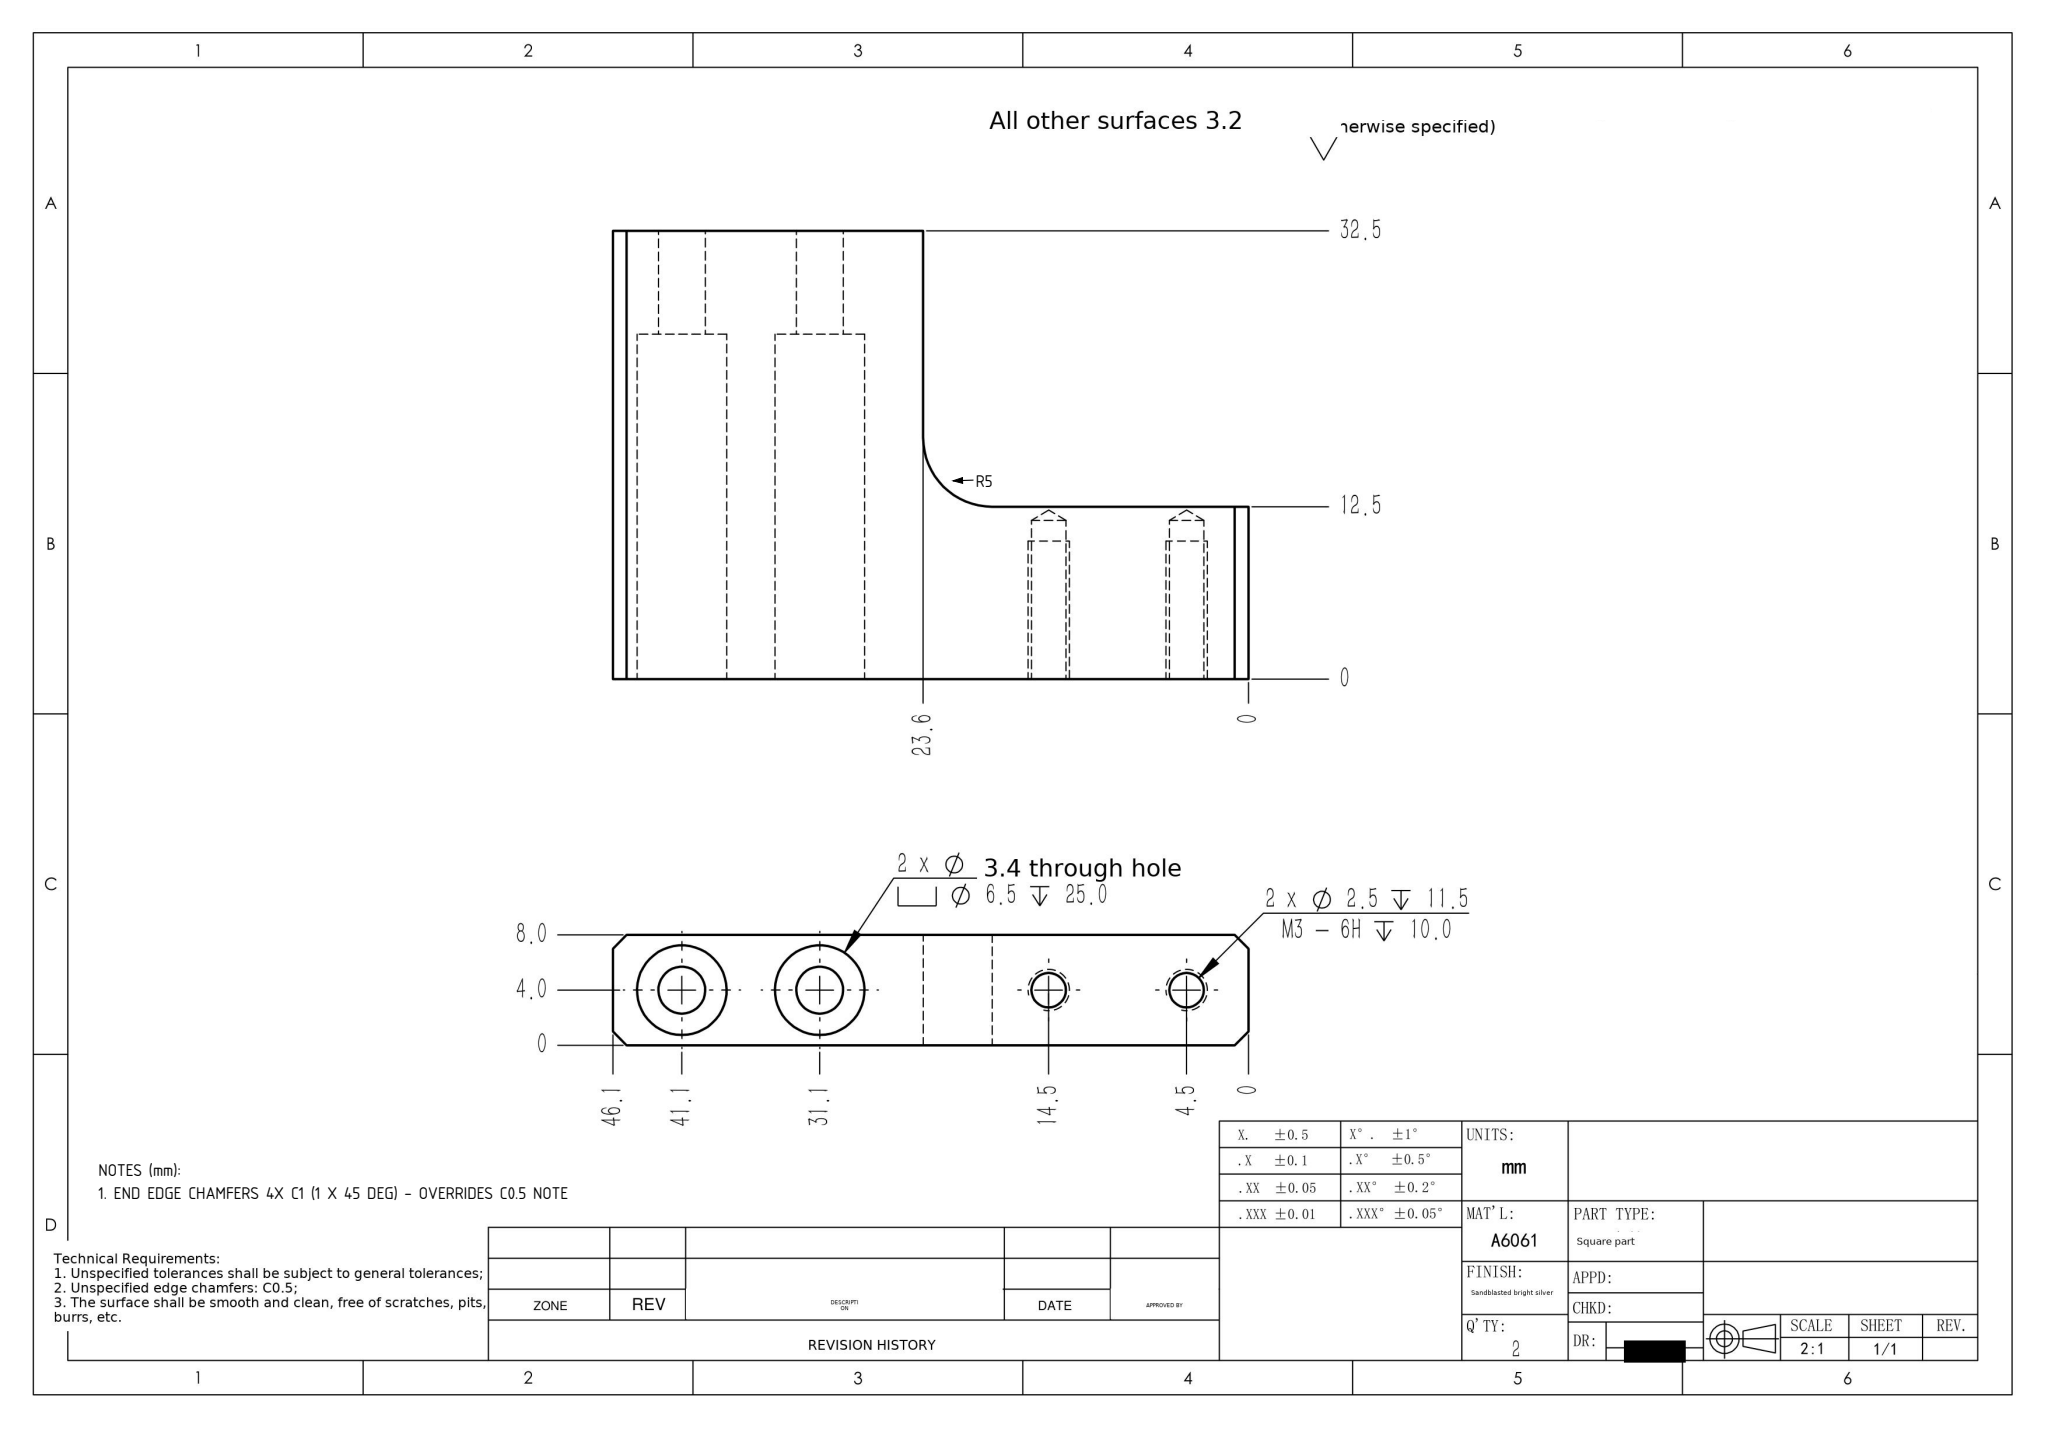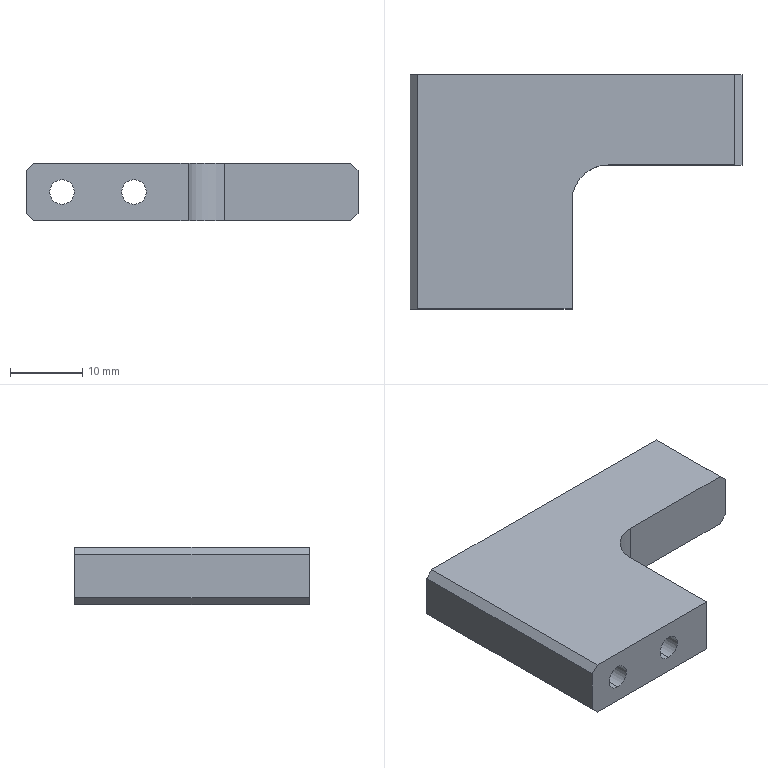Part | SolidWorks | mm | material A6061 | 1 solid | 31 faces | box 46.1 x 32.5 x 8 mm | volume 6297 mm3 | plane 14 | cylinder 13 | cone 4 | commonest cylinder face diameters 2.5 x4 6.5 x4 3.4 x4 10 x1
Drawing notes:
INNER CORNER FILLET R5 AT STEP TRANSITION, TANGENT TO VERTICAL FACE X=22.5 AND HORIZONTAL FACE Y=20.0 (ARC CENTER X27.5, Y15.0 FROM BBOX MIN CORNER), FULL 8.0 THICKNESS | from the solid: cylinders: [10.0, axis z, pos (27.5, 15.0), length 8.0] = R5 concave corner tangent to planes x=22.5 and y=20.0
END EDGE CHAMFERS 4X C1 (1 X 45 DEG) - OVERRIDES C0.5 NOTE | from the solid: inclined_planes: 4 faces at 45/90/45, size 1.0 x L x 1.0, at x=0 (z=0 & z=7, y 0-32.5) and x=45.1 (z=0 & z=7, y 20-32.5)
build123d program:
from build123d import *

# Parameters (mm, degrees)
SKETCH1_W                                       = 46.1
SKETCH1_H                                       = 32.5
BOSS_EXTRUDE1_DEPTH                             = 8
SKETCH2_W                                       = 23.6
SKETCH2_H                                       = 20
CUT_EXTRUDE1_DEPTH                              = 57.969
M3_HEX_SOCKET_HEAD_CAP_SCREW_CBORE1_D           = 3.4
M3_HEX_SOCKET_HEAD_CAP_SCREW_CBORE1_CBORE_D     = 6.5
M3_HEX_SOCKET_HEAD_CAP_SCREW_CBORE1_CBORE_DEPTH = 25
M3_TAPPED_HOLE1_D                               = 2.5
M3_TAPPED_HOLE1_DEPTH                           = 11.5
M3_TAPPED_HOLE1_TIP                             = 0.7511
FILLET1_R                                       = 5
CHAMFER1_SIZE                                   = 1


with BuildPart() as part:
    # Sketch1 → Boss-Extrude1 (new body)
    with BuildSketch(Plane.XY):
        with Locations((23.05, 16.25)):
            Rectangle(SKETCH1_W, SKETCH1_H)
    extrude(amount=BOSS_EXTRUDE1_DEPTH)

    # Sketch2 → Cut-Extrude1 (cut, through all)
    with BuildSketch(Plane.XY.offset(8)):
        with Locations((34.3, 10)):
            Rectangle(SKETCH2_W, SKETCH2_H)
    extrude(amount=-CUT_EXTRUDE1_DEPTH, mode=Mode.SUBTRACT)

    # M3 Hex Socket Head Cap Screw CBORE1 (through all)
    with Locations(Plane(origin=(0, 32.5, 0), x_dir=(1, 0, 0), z_dir=(0, 1, 0))):
        with Locations((5, -4), (15, -4)):
            CounterBoreHole(M3_HEX_SOCKET_HEAD_CAP_SCREW_CBORE1_D / 2, M3_HEX_SOCKET_HEAD_CAP_SCREW_CBORE1_CBORE_D / 2, M3_HEX_SOCKET_HEAD_CAP_SCREW_CBORE1_CBORE_DEPTH)

    # M3 Tapped Hole1
    with Locations(Plane(origin=(0, 32.5, 0), x_dir=(1, 0, 0), z_dir=(0, 1, 0))):
        with Locations((41.6, -4), (31.6, -4)):
            Hole(M3_TAPPED_HOLE1_D / 2, depth=M3_TAPPED_HOLE1_DEPTH)
            with Locations((0, 0, -(M3_TAPPED_HOLE1_DEPTH + M3_TAPPED_HOLE1_TIP / 2))):  # 118° drill point
                Cone(0, M3_TAPPED_HOLE1_D / 2, M3_TAPPED_HOLE1_TIP, mode=Mode.SUBTRACT)

    # Fillet1
    fillet1_edges = [part.edges().sort_by_distance(p)[0] for p in [
        (22.5, 20, 4),
    ]]
    fillet(fillet1_edges, radius=FILLET1_R)

    # Chamfer1
    chamfer1_edges = [part.edges().sort_by_distance(p)[0] for p in [
        (46.1, 26.25, 0),
        (46.1, 26.25, 8),
        (0, 16.25, 8),
        (0, 16.25, 0),
    ]]
    chamfer(chamfer1_edges, length=CHAMFER1_SIZE)


solid = part.part
STEP:
#1=CARTESIAN_POINT('',(41.6,21.,2.75));
#2=VERTEX_POINT('',#1);
#3=CARTESIAN_POINT('',(41.6,21.,5.25));
#4=VERTEX_POINT('',#3);
#5=CARTESIAN_POINT('',(41.6,21.,4.));
#6=DIRECTION('',(0.,1.,0.));
#7=DIRECTION('',(0.,0.,1.));
#8=AXIS2_PLACEMENT_3D('',#5,#6,#7);
#9=CIRCLE('',#8,1.25);
#10=EDGE_CURVE('',#2,#4,#9,.T.);
#11=ORIENTED_EDGE('',*,*,#10,.F.);
#12=CARTESIAN_POINT('',(41.6,32.5,2.75));
#13=VERTEX_POINT('',#12);
#14=CARTESIAN_POINT('',(41.6,32.5,2.75));
#15=DIRECTION('',(0.,1.,0.));
#16=VECTOR('',#15,1000.);
#17=LINE('',#14,#16);
#18=EDGE_CURVE('',#2,#13,#17,.T.);
#19=ORIENTED_EDGE('',*,*,#18,.T.);
#20=CARTESIAN_POINT('',(41.6,32.5,5.25));
#21=VERTEX_POINT('',#20);
#22=CARTESIAN_POINT('',(41.6,32.5,4.));
#23=DIRECTION('',(0.,1.,0.));
#24=DIRECTION('',(0.,0.,1.));
#25=AXIS2_PLACEMENT_3D('',#22,#23,#24);
#26=CIRCLE('',#25,1.25);
#27=EDGE_CURVE('',#13,#21,#26,.T.);
#28=ORIENTED_EDGE('',*,*,#27,.T.);
#29=CARTESIAN_POINT('',(41.6,32.5,5.25));
#30=DIRECTION('',(0.,1.,0.));
#31=VECTOR('',#30,1000.);
#32=LINE('',#29,#31);
#33=EDGE_CURVE('',#4,#21,#32,.T.);
#34=ORIENTED_EDGE('',*,*,#33,.F.);
#35=EDGE_LOOP('',(#11,#19,#28,#34));
#36=FACE_OUTER_BOUND('',#35,.T.);
#37=CARTESIAN_POINT('',(41.6,32.5,4.));
#38=DIRECTION('',(0.,1.,0.));
#39=DIRECTION('',(0.,0.,1.));
#40=AXIS2_PLACEMENT_3D('',#37,#38,#39);
#41=CYLINDRICAL_SURFACE('',#40,1.25);
#42=ADVANCED_FACE('',(#36),#41,.F.);
#43=CARTESIAN_POINT('',(41.6,20.249,4.));
#44=VERTEX_POINT('',#43);
#45=CARTESIAN_POINT('',(41.6,21.,5.25));
#46=DIRECTION('',(0.,0.515,0.8572));
#47=VECTOR('',#46,1000.);
#48=LINE('',#45,#47);
#49=EDGE_CURVE('',#44,#4,#48,.T.);
#50=ORIENTED_EDGE('',*,*,#49,.F.);
#51=CARTESIAN_POINT('',(41.6,21.,2.75));
#52=DIRECTION('',(0.,0.515,-0.8572));
#53=VECTOR('',#52,1000.);
#54=LINE('',#51,#53);
#55=EDGE_CURVE('',#44,#2,#54,.T.);
#56=ORIENTED_EDGE('',*,*,#55,.T.);
#57=ORIENTED_EDGE('',*,*,#10,.T.);
#58=EDGE_LOOP('',(#50,#56,#57));
#59=FACE_OUTER_BOUND('',#58,.T.);
#60=CARTESIAN_POINT('',(41.6,21.,4.));
#61=DIRECTION('',(0.,1.,0.));
#62=DIRECTION('',(0.,0.,1.));
#63=AXIS2_PLACEMENT_3D('',#60,#61,#62);
#64=CONICAL_SURFACE('',#63,1.25,1.03);
#65=ADVANCED_FACE('',(#59),#64,.F.);
#66=CARTESIAN_POINT('',(31.6,21.,2.75));
#67=VERTEX_POINT('',#66);
#68=CARTESIAN_POINT('',(31.6,21.,5.25));
#69=VERTEX_POINT('',#68);
#70=CARTESIAN_POINT('',(31.6,21.,4.));
#71=DIRECTION('',(0.,1.,0.));
#72=DIRECTION('',(0.,0.,1.));
#73=AXIS2_PLACEMENT_3D('',#70,#71,#72);
#74=CIRCLE('',#73,1.25);
#75=EDGE_CURVE('',#67,#69,#74,.T.);
#76=ORIENTED_EDGE('',*,*,#75,.F.);
#77=CARTESIAN_POINT('',(31.6,32.5,2.75));
#78=VERTEX_POINT('',#77);
#79=CARTESIAN_POINT('',(31.6,32.5,2.75));
#80=DIRECTION('',(0.,1.,0.));
#81=VECTOR('',#80,1000.);
#82=LINE('',#79,#81);
#83=EDGE_CURVE('',#67,#78,#82,.T.);
#84=ORIENTED_EDGE('',*,*,#83,.T.);
#85=CARTESIAN_POINT('',(31.6,32.5,5.25));
#86=VERTEX_POINT('',#85);
#87=CARTESIAN_POINT('',(31.6,32.5,4.));
#88=DIRECTION('',(0.,1.,0.));
#89=DIRECTION('',(0.,0.,1.));
#90=AXIS2_PLACEMENT_3D('',#87,#88,#89);
#91=CIRCLE('',#90,1.25);
#92=EDGE_CURVE('',#78,#86,#91,.T.);
#93=ORIENTED_EDGE('',*,*,#92,.T.);
#94=CARTESIAN_POINT('',(31.6,32.5,5.25));
#95=DIRECTION('',(0.,1.,0.));
#96=VECTOR('',#95,1000.);
#97=LINE('',#94,#96);
#98=EDGE_CURVE('',#69,#86,#97,.T.);
#99=ORIENTED_EDGE('',*,*,#98,.F.);
#100=EDGE_LOOP('',(#76,#84,#93,#99));
#101=FACE_OUTER_BOUND('',#100,.T.);
#102=CARTESIAN_POINT('',(31.6,32.5,4.));
#103=DIRECTION('',(0.,1.,0.));
#104=DIRECTION('',(0.,0.,1.));
#105=AXIS2_PLACEMENT_3D('',#102,#103,#104);
#106=CYLINDRICAL_SURFACE('',#105,1.25);
#107=ADVANCED_FACE('',(#101),#106,.F.);
#108=CARTESIAN_POINT('',(31.6,20.249,4.));
#109=VERTEX_POINT('',#108);
#110=CARTESIAN_POINT('',(31.6,21.,5.25));
#111=DIRECTION('',(0.,0.515,0.8572));
#112=VECTOR('',#111,1000.);
#113=LINE('',#110,#112);
#114=EDGE_CURVE('',#109,#69,#113,.T.);
#115=ORIENTED_EDGE('',*,*,#114,.F.);
#116=CARTESIAN_POINT('',(31.6,21.,2.75));
#117=DIRECTION('',(0.,0.515,-0.8572));
#118=VECTOR('',#117,1000.);
#119=LINE('',#116,#118);
#120=EDGE_CURVE('',#109,#67,#119,.T.);
#121=ORIENTED_EDGE('',*,*,#120,.T.);
#122=ORIENTED_EDGE('',*,*,#75,.T.);
#123=EDGE_LOOP('',(#115,#121,#122));
#124=FACE_OUTER_BOUND('',#123,.T.);
#125=CARTESIAN_POINT('',(31.6,21.,4.));
#126=DIRECTION('',(0.,1.,0.));
#127=DIRECTION('',(0.,0.,1.));
#128=AXIS2_PLACEMENT_3D('',#125,#126,#127);
#129=CONICAL_SURFACE('',#128,1.25,1.03);
#130=ADVANCED_FACE('',(#124),#129,.F.);
#131=CARTESIAN_POINT('',(5.,7.5,0.75));
#132=VERTEX_POINT('',#131);
#133=CARTESIAN_POINT('',(5.,7.5,7.25));
#134=VERTEX_POINT('',#133);
#135=CARTESIAN_POINT('',(5.,7.5,4.));
#136=DIRECTION('',(0.,1.,0.));
#137=DIRECTION('',(0.,0.,1.));
#138=AXIS2_PLACEMENT_3D('',#135,#136,#137);
#139=CIRCLE('',#138,3.25);
#140=EDGE_CURVE('',#132,#134,#139,.T.);
#141=ORIENTED_EDGE('',*,*,#140,.F.);
#142=CARTESIAN_POINT('',(5.,32.5,0.75));
#143=VERTEX_POINT('',#142);
#144=CARTESIAN_POINT('',(5.,32.5,0.75));
#145=DIRECTION('',(0.,1.,0.));
#146=VECTOR('',#145,1000.);
#147=LINE('',#144,#146);
#148=EDGE_CURVE('',#132,#143,#147,.T.);
#149=ORIENTED_EDGE('',*,*,#148,.T.);
#150=CARTESIAN_POINT('',(5.,32.5,7.25));
#151=VERTEX_POINT('',#150);
#152=CARTESIAN_POINT('',(5.,32.5,4.));
#153=DIRECTION('',(0.,1.,0.));
#154=DIRECTION('',(0.,0.,1.));
#155=AXIS2_PLACEMENT_3D('',#152,#153,#154);
#156=CIRCLE('',#155,3.25);
#157=EDGE_CURVE('',#143,#151,#156,.T.);
#158=ORIENTED_EDGE('',*,*,#157,.T.);
#159=CARTESIAN_POINT('',(5.,32.5,7.25));
#160=DIRECTION('',(0.,1.,0.));
#161=VECTOR('',#160,1000.);
#162=LINE('',#159,#161);
#163=EDGE_CURVE('',#134,#151,#162,.T.);
#164=ORIENTED_EDGE('',*,*,#163,.F.);
#165=EDGE_LOOP('',(#141,#149,#158,#164));
#166=FACE_OUTER_BOUND('',#165,.T.);
#167=CARTESIAN_POINT('',(5.,32.5,4.));
#168=DIRECTION('',(0.,1.,0.));
#169=DIRECTION('',(0.,0.,1.));
#170=AXIS2_PLACEMENT_3D('',#167,#168,#169);
#171=CYLINDRICAL_SURFACE('',#170,3.25);
#172=ADVANCED_FACE('',(#166),#171,.F.);
#173=CARTESIAN_POINT('',(5.,0.,2.3));
#174=VERTEX_POINT('',#173);
#175=CARTESIAN_POINT('',(5.,0.,5.7));
#176=VERTEX_POINT('',#175);
#177=CARTESIAN_POINT('',(5.,0.,4.));
#178=DIRECTION('',(0.,1.,0.));
#179=DIRECTION('',(0.,0.,1.));
#180=AXIS2_PLACEMENT_3D('',#177,#178,#179);
#181=CIRCLE('',#180,1.7);
#182=EDGE_CURVE('',#174,#176,#181,.T.);
#183=ORIENTED_EDGE('',*,*,#182,.F.);
#184=CARTESIAN_POINT('',(5.,7.5,2.3));
#185=VERTEX_POINT('',#184);
#186=CARTESIAN_POINT('',(5.,32.5,2.3));
#187=DIRECTION('',(0.,1.,0.));
#188=VECTOR('',#187,1000.);
#189=LINE('',#186,#188);
#190=EDGE_CURVE('',#174,#185,#189,.T.);
#191=ORIENTED_EDGE('',*,*,#190,.T.);
#192=CARTESIAN_POINT('',(5.,7.5,5.7));
#193=VERTEX_POINT('',#192);
#194=CARTESIAN_POINT('',(5.,7.5,4.));
#195=DIRECTION('',(0.,1.,0.));
#196=DIRECTION('',(0.,0.,1.));
#197=AXIS2_PLACEMENT_3D('',#194,#195,#196);
#198=CIRCLE('',#197,1.7);
#199=EDGE_CURVE('',#185,#193,#198,.T.);
#200=ORIENTED_EDGE('',*,*,#199,.T.);
#201=CARTESIAN_POINT('',(5.,32.5,5.7));
#202=DIRECTION('',(0.,1.,0.));
#203=VECTOR('',#202,1000.);
#204=LINE('',#201,#203);
#205=EDGE_CURVE('',#176,#193,#204,.T.);
#206=ORIENTED_EDGE('',*,*,#205,.F.);
#207=EDGE_LOOP('',(#183,#191,#200,#206));
#208=FACE_OUTER_BOUND('',#207,.T.);
#209=CARTESIAN_POINT('',(5.,32.5,4.));
#210=DIRECTION('',(0.,1.,0.));
#211=DIRECTION('',(0.,0.,1.));
#212=AXIS2_PLACEMENT_3D('',#209,#210,#211);
#213=CYLINDRICAL_SURFACE('',#212,1.7);
#214=ADVANCED_FACE('',(#208),#213,.F.);
#215=CARTESIAN_POINT('',(15.,7.5,0.75));
#216=VERTEX_POINT('',#215);
#217=CARTESIAN_POINT('',(15.,7.5,7.25));
#218=VERTEX_POINT('',#217);
#219=CARTESIAN_POINT('',(15.,7.5,4.));
#220=DIRECTION('',(0.,1.,0.));
#221=DIRECTION('',(0.,0.,1.));
#222=AXIS2_PLACEMENT_3D('',#219,#220,#221);
#223=CIRCLE('',#222,3.25);
#224=EDGE_CURVE('',#216,#218,#223,.T.);
#225=ORIENTED_EDGE('',*,*,#224,.F.);
#226=CARTESIAN_POINT('',(15.,32.5,0.75));
#227=VERTEX_POINT('',#226);
#228=CARTESIAN_POINT('',(15.,32.5,0.75));
#229=DIRECTION('',(0.,1.,0.));
#230=VECTOR('',#229,1000.);
#231=LINE('',#228,#230);
#232=EDGE_CURVE('',#216,#227,#231,.T.);
#233=ORIENTED_EDGE('',*,*,#232,.T.);
#234=CARTESIAN_POINT('',(15.,32.5,7.25));
#235=VERTEX_POINT('',#234);
#236=CARTESIAN_POINT('',(15.,32.5,4.));
#237=DIRECTION('',(0.,1.,0.));
#238=DIRECTION('',(0.,0.,1.));
#239=AXIS2_PLACEMENT_3D('',#236,#237,#238);
#240=CIRCLE('',#239,3.25);
#241=EDGE_CURVE('',#227,#235,#240,.T.);
#242=ORIENTED_EDGE('',*,*,#241,.T.);
#243=CARTESIAN_POINT('',(15.,32.5,7.25));
#244=DIRECTION('',(0.,1.,0.));
#245=VECTOR('',#244,1000.);
#246=LINE('',#243,#245);
#247=EDGE_CURVE('',#218,#235,#246,.T.);
#248=ORIENTED_EDGE('',*,*,#247,.F.);
#249=EDGE_LOOP('',(#225,#233,#242,#248));
#250=FACE_OUTER_BOUND('',#249,.T.);
#251=CARTESIAN_POINT('',(15.,32.5,4.));
#252=DIRECTION('',(0.,1.,0.));
#253=DIRECTION('',(0.,0.,1.));
#254=AXIS2_PLACEMENT_3D('',#251,#252,#253);
#255=CYLINDRICAL_SURFACE('',#254,3.25);
#256=ADVANCED_FACE('',(#250),#255,.F.);
#257=CARTESIAN_POINT('',(15.,0.,2.3));
#258=VERTEX_POINT('',#257);
#259=CARTESIAN_POINT('',(15.,0.,5.7));
#260=VERTEX_POINT('',#259);
#261=CARTESIAN_POINT('',(15.,0.,4.));
#262=DIRECTION('',(0.,1.,0.));
#263=DIRECTION('',(0.,0.,1.));
#264=AXIS2_PLACEMENT_3D('',#261,#262,#263);
#265=CIRCLE('',#264,1.7);
#266=EDGE_CURVE('',#258,#260,#265,.T.);
#267=ORIENTED_EDGE('',*,*,#266,.F.);
#268=CARTESIAN_POINT('',(15.,7.5,2.3));
#269=VERTEX_POINT('',#268);
#270=CARTESIAN_POINT('',(15.,32.5,2.3));
#271=DIRECTION('',(0.,1.,0.));
#272=VECTOR('',#271,1000.);
#273=LINE('',#270,#272);
#274=EDGE_CURVE('',#258,#269,#273,.T.);
#275=ORIENTED_EDGE('',*,*,#274,.T.);
#276=CARTESIAN_POINT('',(15.,7.5,5.7));
#277=VERTEX_POINT('',#276);
#278=CARTESIAN_POINT('',(15.,7.5,4.));
#279=DIRECTION('',(0.,1.,0.));
#280=DIRECTION('',(0.,0.,1.));
#281=AXIS2_PLACEMENT_3D('',#278,#279,#280);
#282=CIRCLE('',#281,1.7);
#283=EDGE_CURVE('',#269,#277,#282,.T.);
#284=ORIENTED_EDGE('',*,*,#283,.T.);
#285=CARTESIAN_POINT('',(15.,32.5,5.7));
#286=DIRECTION('',(0.,1.,0.));
#287=VECTOR('',#286,1000.);
#288=LINE('',#285,#287);
#289=EDGE_CURVE('',#260,#277,#288,.T.);
#290=ORIENTED_EDGE('',*,*,#289,.F.);
#291=EDGE_LOOP('',(#267,#275,#284,#290));
#292=FACE_OUTER_BOUND('',#291,.T.);
#293=CARTESIAN_POINT('',(15.,32.5,4.));
#294=DIRECTION('',(0.,1.,0.));
#295=DIRECTION('',(0.,0.,1.));
#296=AXIS2_PLACEMENT_3D('',#293,#294,#295);
#297=CYLINDRICAL_SURFACE('',#296,1.7);
#298=ADVANCED_FACE('',(#292),#297,.F.);
#299=CARTESIAN_POINT('',(0.,0.,7.));
#300=VERTEX_POINT('',#299);
#301=CARTESIAN_POINT('',(0.,0.,1.));
#302=VERTEX_POINT('',#301);
#303=CARTESIAN_POINT('',(0.,0.,8.));
#304=DIRECTION('',(0.,0.,-1.));
#305=VECTOR('',#304,1000.);
#306=LINE('',#303,#305);
#307=EDGE_CURVE('',#300,#302,#306,.T.);
#308=ORIENTED_EDGE('',*,*,#307,.F.);
#309=CARTESIAN_POINT('',(0.,32.5,7.));
#310=VERTEX_POINT('',#309);
#311=CARTESIAN_POINT('',(0.,0.,7.));
#312=DIRECTION('',(0.,1.,0.));
#313=VECTOR('',#312,1000.);
#314=LINE('',#311,#313);
#315=EDGE_CURVE('',#300,#310,#314,.T.);
#316=ORIENTED_EDGE('',*,*,#315,.T.);
#317=CARTESIAN_POINT('',(0.,32.5,1.));
#318=VERTEX_POINT('',#317);
#319=CARTESIAN_POINT('',(0.,32.5,8.));
#320=DIRECTION('',(0.,0.,-1.));
#321=VECTOR('',#320,1000.);
#322=LINE('',#319,#321);
#323=EDGE_CURVE('',#310,#318,#322,.T.);
#324=ORIENTED_EDGE('',*,*,#323,.T.);
#325=CARTESIAN_POINT('',(0.,0.,1.));
#326=DIRECTION('',(0.,-1.,0.));
#327=VECTOR('',#326,1000.);
#328=LINE('',#325,#327);
#329=EDGE_CURVE('',#318,#302,#328,.T.);
#330=ORIENTED_EDGE('',*,*,#329,.T.);
#331=EDGE_LOOP('',(#308,#316,#324,#330));
#332=FACE_OUTER_BOUND('',#331,.T.);
#333=CARTESIAN_POINT('',(0.,0.,8.));
#334=DIRECTION('',(1.,0.,0.));
#335=DIRECTION('',(0.,0.,-1.));
#336=AXIS2_PLACEMENT_3D('',#333,#334,#335);
#337=PLANE('',#336);
#338=ADVANCED_FACE('',(#332),#337,.F.);
#339=CARTESIAN_POINT('',(5.,0.,4.));
#340=DIRECTION('',(0.,1.,0.));
#341=DIRECTION('',(0.,0.,1.));
#342=AXIS2_PLACEMENT_3D('',#339,#340,#341);
#343=CIRCLE('',#342,1.7);
#344=EDGE_CURVE('',#176,#174,#343,.T.);
#345=ORIENTED_EDGE('',*,*,#344,.T.);
#346=ORIENTED_EDGE('',*,*,#182,.T.);
#347=EDGE_LOOP('',(#345,#346));
#348=FACE_BOUND('',#347,.T.);
#349=CARTESIAN_POINT('',(15.,0.,4.));
#350=DIRECTION('',(0.,1.,0.));
#351=DIRECTION('',(0.,0.,1.));
#352=AXIS2_PLACEMENT_3D('',#349,#350,#351);
#353=CIRCLE('',#352,1.7);
#354=EDGE_CURVE('',#260,#258,#353,.T.);
#355=ORIENTED_EDGE('',*,*,#354,.T.);
#356=ORIENTED_EDGE('',*,*,#266,.T.);
#357=EDGE_LOOP('',(#355,#356));
#358=FACE_BOUND('',#357,.T.);
#359=CARTESIAN_POINT('',(1.,0.,8.));
#360=VERTEX_POINT('',#359);
#361=CARTESIAN_POINT('',(22.5,-0.,8.));
#362=VERTEX_POINT('',#361);
#363=CARTESIAN_POINT('',(0.,0.,8.));
#364=DIRECTION('',(1.,0.,0.));
#365=VECTOR('',#364,1000.);
#366=LINE('',#363,#365);
#367=EDGE_CURVE('',#360,#362,#366,.T.);
#368=ORIENTED_EDGE('',*,*,#367,.F.);
#369=CARTESIAN_POINT('',(1.,0.,8.));
#370=DIRECTION('',(-0.7071,0.,-0.7071));
#371=VECTOR('',#370,1000.);
#372=LINE('',#369,#371);
#373=EDGE_CURVE('',#360,#300,#372,.T.);
#374=ORIENTED_EDGE('',*,*,#373,.T.);
#375=ORIENTED_EDGE('',*,*,#307,.T.);
#376=CARTESIAN_POINT('',(1.,0.,0.));
#377=VERTEX_POINT('',#376);
#378=CARTESIAN_POINT('',(0.,0.,1.));
#379=DIRECTION('',(0.7071,0.,-0.7071));
#380=VECTOR('',#379,1000.);
#381=LINE('',#378,#380);
#382=EDGE_CURVE('',#302,#377,#381,.T.);
#383=ORIENTED_EDGE('',*,*,#382,.T.);
#384=CARTESIAN_POINT('',(22.5,-0.,0.));
#385=VERTEX_POINT('',#384);
#386=CARTESIAN_POINT('',(0.,0.,0.));
#387=DIRECTION('',(1.,0.,0.));
#388=VECTOR('',#387,1000.);
#389=LINE('',#386,#388);
#390=EDGE_CURVE('',#377,#385,#389,.T.);
#391=ORIENTED_EDGE('',*,*,#390,.T.);
#392=CARTESIAN_POINT('',(22.5,-0.,0.));
#393=DIRECTION('',(0.,0.,1.));
#394=VECTOR('',#393,1000.);
#395=LINE('',#392,#394);
#396=EDGE_CURVE('',#385,#362,#395,.T.);
#397=ORIENTED_EDGE('',*,*,#396,.T.);
#398=EDGE_LOOP('',(#368,#374,#375,#383,#391,#397));
#399=FACE_OUTER_BOUND('',#398,.T.);
#400=CARTESIAN_POINT('',(0.,0.,8.));
#401=DIRECTION('',(0.,1.,0.));
#402=DIRECTION('',(0.,0.,1.));
#403=AXIS2_PLACEMENT_3D('',#400,#401,#402);
#404=PLANE('',#403);
#405=ADVANCED_FACE('',(#348,#358,#399),#404,.F.);
#406=CARTESIAN_POINT('',(46.1,32.5,7.));
#407=VERTEX_POINT('',#406);
#408=CARTESIAN_POINT('',(46.1,32.5,1.));
#409=VERTEX_POINT('',#408);
#410=CARTESIAN_POINT('',(46.1,32.5,8.));
#411=DIRECTION('',(0.,0.,-1.));
#412=VECTOR('',#411,1000.);
#413=LINE('',#410,#412);
#414=EDGE_CURVE('',#407,#409,#413,.T.);
#415=ORIENTED_EDGE('',*,*,#414,.F.);
#416=CARTESIAN_POINT('',(46.1,20.,7.));
#417=VERTEX_POINT('',#416);
#418=CARTESIAN_POINT('',(46.1,0.,7.));
#419=DIRECTION('',(0.,-1.,0.));
#420=VECTOR('',#419,1000.);
#421=LINE('',#418,#420);
#422=EDGE_CURVE('',#407,#417,#421,.T.);
#423=ORIENTED_EDGE('',*,*,#422,.T.);
#424=CARTESIAN_POINT('',(46.1,20.,1.));
#425=VERTEX_POINT('',#424);
#426=CARTESIAN_POINT('',(46.1,20.,0.));
#427=DIRECTION('',(0.,0.,1.));
#428=VECTOR('',#427,1000.);
#429=LINE('',#426,#428);
#430=EDGE_CURVE('',#425,#417,#429,.T.);
#431=ORIENTED_EDGE('',*,*,#430,.F.);
#432=CARTESIAN_POINT('',(46.1,32.5,1.));
#433=DIRECTION('',(0.,1.,0.));
#434=VECTOR('',#433,1000.);
#435=LINE('',#432,#434);
#436=EDGE_CURVE('',#425,#409,#435,.T.);
#437=ORIENTED_EDGE('',*,*,#436,.T.);
#438=EDGE_LOOP('',(#415,#423,#431,#437));
#439=FACE_OUTER_BOUND('',#438,.T.);
#440=CARTESIAN_POINT('',(46.1,0.,8.));
#441=DIRECTION('',(-1.,0.,0.));
#442=DIRECTION('',(0.,0.,1.));
#443=AXIS2_PLACEMENT_3D('',#440,#441,#442);
#444=PLANE('',#443);
#445=ADVANCED_FACE('',(#439),#444,.F.);
#446=CARTESIAN_POINT('',(41.6,32.5,4.));
#447=DIRECTION('',(0.,1.,0.));
#448=DIRECTION('',(0.,0.,1.));
#449=AXIS2_PLACEMENT_3D('',#446,#447,#448);
#450=CIRCLE('',#449,1.25);
#451=EDGE_CURVE('',#21,#13,#450,.T.);
#452=ORIENTED_EDGE('',*,*,#451,.F.);
#453=ORIENTED_EDGE('',*,*,#27,.F.);
#454=EDGE_LOOP('',(#452,#453));
#455=FACE_BOUND('',#454,.T.);
#456=CARTESIAN_POINT('',(31.6,32.5,4.));
#457=DIRECTION('',(0.,1.,0.));
#458=DIRECTION('',(0.,0.,1.));
#459=AXIS2_PLACEMENT_3D('',#456,#457,#458);
#460=CIRCLE('',#459,1.25);
#461=EDGE_CURVE('',#86,#78,#460,.T.);
#462=ORIENTED_EDGE('',*,*,#461,.F.);
#463=ORIENTED_EDGE('',*,*,#92,.F.);
#464=EDGE_LOOP('',(#462,#463));
#465=FACE_BOUND('',#464,.T.);
#466=CARTESIAN_POINT('',(5.,32.5,4.));
#467=DIRECTION('',(0.,1.,0.));
#468=DIRECTION('',(0.,0.,1.));
#469=AXIS2_PLACEMENT_3D('',#466,#467,#468);
#470=CIRCLE('',#469,3.25);
#471=EDGE_CURVE('',#151,#143,#470,.T.);
#472=ORIENTED_EDGE('',*,*,#471,.F.);
#473=ORIENTED_EDGE('',*,*,#157,.F.);
#474=EDGE_LOOP('',(#472,#473));
#475=FACE_BOUND('',#474,.T.);
#476=CARTESIAN_POINT('',(15.,32.5,4.));
#477=DIRECTION('',(0.,1.,0.));
#478=DIRECTION('',(0.,0.,1.));
#479=AXIS2_PLACEMENT_3D('',#476,#477,#478);
#480=CIRCLE('',#479,3.25);
#481=EDGE_CURVE('',#235,#227,#480,.T.);
#482=ORIENTED_EDGE('',*,*,#481,.F.);
#483=ORIENTED_EDGE('',*,*,#241,.F.);
#484=EDGE_LOOP('',(#482,#483));
#485=FACE_BOUND('',#484,.T.);
#486=CARTESIAN_POINT('',(45.1,32.5,8.));
#487=VERTEX_POINT('',#486);
#488=CARTESIAN_POINT('',(1.,32.5,8.));
#489=VERTEX_POINT('',#488);
#490=CARTESIAN_POINT('',(0.,32.5,8.));
#491=DIRECTION('',(-1.,0.,0.));
#492=VECTOR('',#491,1000.);
#493=LINE('',#490,#492);
#494=EDGE_CURVE('',#487,#489,#493,.T.);
#495=ORIENTED_EDGE('',*,*,#494,.F.);
#496=CARTESIAN_POINT('',(45.1,32.5,8.));
#497=DIRECTION('',(0.7071,0.,-0.7071));
#498=VECTOR('',#497,1000.);
#499=LINE('',#496,#498);
#500=EDGE_CURVE('',#487,#407,#499,.T.);
#501=ORIENTED_EDGE('',*,*,#500,.T.);
#502=ORIENTED_EDGE('',*,*,#414,.T.);
#503=CARTESIAN_POINT('',(45.1,32.5,0.));
#504=VERTEX_POINT('',#503);
#505=CARTESIAN_POINT('',(46.1,32.5,1.));
#506=DIRECTION('',(-0.7071,0.,-0.7071));
#507=VECTOR('',#506,1000.);
#508=LINE('',#505,#507);
#509=EDGE_CURVE('',#409,#504,#508,.T.);
#510=ORIENTED_EDGE('',*,*,#509,.T.);
#511=CARTESIAN_POINT('',(1.,32.5,0.));
#512=VERTEX_POINT('',#511);
#513=CARTESIAN_POINT('',(0.,32.5,0.));
#514=DIRECTION('',(-1.,0.,0.));
#515=VECTOR('',#514,1000.);
#516=LINE('',#513,#515);
#517=EDGE_CURVE('',#504,#512,#516,.T.);
#518=ORIENTED_EDGE('',*,*,#517,.T.);
#519=CARTESIAN_POINT('',(0.,32.5,1.));
#520=DIRECTION('',(-0.7071,0.,0.7071));
#521=VECTOR('',#520,1000.);
#522=LINE('',#519,#521);
#523=EDGE_CURVE('',#512,#318,#522,.T.);
#524=ORIENTED_EDGE('',*,*,#523,.T.);
#525=ORIENTED_EDGE('',*,*,#323,.F.);
#526=CARTESIAN_POINT('',(1.,32.5,8.));
#527=DIRECTION('',(0.7071,0.,0.7071));
#528=VECTOR('',#527,1000.);
#529=LINE('',#526,#528);
#530=EDGE_CURVE('',#310,#489,#529,.T.);
#531=ORIENTED_EDGE('',*,*,#530,.T.);
#532=EDGE_LOOP('',(#495,#501,#502,#510,#518,#524,#525,#531));
#533=FACE_OUTER_BOUND('',#532,.T.);
#534=CARTESIAN_POINT('',(0.,32.5,8.));
#535=DIRECTION('',(0.,-1.,0.));
#536=DIRECTION('',(0.,0.,-1.));
#537=AXIS2_PLACEMENT_3D('',#534,#535,#536);
#538=PLANE('',#537);
#539=ADVANCED_FACE('',(#455,#465,#475,#485,#533),#538,.F.);
#540=CARTESIAN_POINT('',(45.1,20.,8.));
#541=VERTEX_POINT('',#540);
#542=CARTESIAN_POINT('',(27.5,20.,8.));
#543=VERTEX_POINT('',#542);
#544=CARTESIAN_POINT('',(46.1,20.,8.));
#545=DIRECTION('',(-1.,-0.,0.));
#546=VECTOR('',#545,1000.);
#547=LINE('',#544,#546);
#548=EDGE_CURVE('',#541,#543,#547,.T.);
#549=ORIENTED_EDGE('',*,*,#548,.F.);
#550=CARTESIAN_POINT('',(45.1,0.,8.));
#551=DIRECTION('',(0.,1.,0.));
#552=VECTOR('',#551,1000.);
#553=LINE('',#550,#552);
#554=EDGE_CURVE('',#541,#487,#553,.T.);
#555=ORIENTED_EDGE('',*,*,#554,.T.);
#556=ORIENTED_EDGE('',*,*,#494,.T.);
#557=CARTESIAN_POINT('',(1.,0.,8.));
#558=DIRECTION('',(0.,-1.,0.));
#559=VECTOR('',#558,1000.);
#560=LINE('',#557,#559);
#561=EDGE_CURVE('',#489,#360,#560,.T.);
#562=ORIENTED_EDGE('',*,*,#561,.T.);
#563=ORIENTED_EDGE('',*,*,#367,.T.);
#564=CARTESIAN_POINT('',(22.5,15.,8.));
#565=VERTEX_POINT('',#564);
#566=CARTESIAN_POINT('',(22.5,-0.,8.));
#567=DIRECTION('',(0.,-1.,0.));
#568=VECTOR('',#567,1000.);
#569=LINE('',#566,#568);
#570=EDGE_CURVE('',#565,#362,#569,.T.);
#571=ORIENTED_EDGE('',*,*,#570,.F.);
#572=CARTESIAN_POINT('',(27.5,15.,8.));
#573=DIRECTION('',(0.,0.,-1.));
#574=DIRECTION('',(-1.,0.,0.));
#575=AXIS2_PLACEMENT_3D('',#572,#573,#574);
#576=CIRCLE('',#575,5.);
#577=EDGE_CURVE('',#565,#543,#576,.T.);
#578=ORIENTED_EDGE('',*,*,#577,.T.);
#579=EDGE_LOOP('',(#549,#555,#556,#562,#563,#571,#578));
#580=FACE_OUTER_BOUND('',#579,.T.);
#581=CARTESIAN_POINT('',(0.,0.,8.));
#582=DIRECTION('',(0.,0.,-1.));
#583=DIRECTION('',(-1.,0.,0.));
#584=AXIS2_PLACEMENT_3D('',#581,#582,#583);
#585=PLANE('',#584);
#586=ADVANCED_FACE('',(#580),#585,.F.);
#587=ORIENTED_EDGE('',*,*,#517,.F.);
#588=CARTESIAN_POINT('',(45.1,20.,0.));
#589=VERTEX_POINT('',#588);
#590=CARTESIAN_POINT('',(45.1,20.,0.));
#591=DIRECTION('',(0.,-1.,0.));
#592=VECTOR('',#591,1000.);
#593=LINE('',#590,#592);
#594=EDGE_CURVE('',#504,#589,#593,.T.);
#595=ORIENTED_EDGE('',*,*,#594,.T.);
#596=CARTESIAN_POINT('',(27.5,20.,0.));
#597=VERTEX_POINT('',#596);
#598=CARTESIAN_POINT('',(46.1,20.,0.));
#599=DIRECTION('',(-1.,-0.,0.));
#600=VECTOR('',#599,1000.);
#601=LINE('',#598,#600);
#602=EDGE_CURVE('',#589,#597,#601,.T.);
#603=ORIENTED_EDGE('',*,*,#602,.T.);
#604=CARTESIAN_POINT('',(22.5,15.,0.));
#605=VERTEX_POINT('',#604);
#606=CARTESIAN_POINT('',(27.5,15.,0.));
#607=DIRECTION('',(0.,0.,1.));
#608=DIRECTION('',(-1.,0.,0.));
#609=AXIS2_PLACEMENT_3D('',#606,#607,#608);
#610=CIRCLE('',#609,5.);
#611=EDGE_CURVE('',#597,#605,#610,.T.);
#612=ORIENTED_EDGE('',*,*,#611,.T.);
#613=CARTESIAN_POINT('',(22.5,-0.,0.));
#614=DIRECTION('',(0.,-1.,0.));
#615=VECTOR('',#614,1000.);
#616=LINE('',#613,#615);
#617=EDGE_CURVE('',#605,#385,#616,.T.);
#618=ORIENTED_EDGE('',*,*,#617,.T.);
#619=ORIENTED_EDGE('',*,*,#390,.F.);
#620=CARTESIAN_POINT('',(1.,32.5,0.));
#621=DIRECTION('',(0.,1.,0.));
#622=VECTOR('',#621,1000.);
#623=LINE('',#620,#622);
#624=EDGE_CURVE('',#377,#512,#623,.T.);
#625=ORIENTED_EDGE('',*,*,#624,.T.);
#626=EDGE_LOOP('',(#587,#595,#603,#612,#618,#619,#625));
#627=FACE_OUTER_BOUND('',#626,.T.);
#628=CARTESIAN_POINT('',(0.,0.,0.));
#629=DIRECTION('',(0.,0.,-1.));
#630=DIRECTION('',(-1.,0.,0.));
#631=AXIS2_PLACEMENT_3D('',#628,#629,#630);
#632=PLANE('',#631);
#633=ADVANCED_FACE('',(#627),#632,.T.);
#634=ORIENTED_EDGE('',*,*,#617,.F.);
#635=CARTESIAN_POINT('',(22.5,15.,8.));
#636=DIRECTION('',(0.,0.,1.));
#637=VECTOR('',#636,1000.);
#638=LINE('',#635,#637);
#639=EDGE_CURVE('',#605,#565,#638,.T.);
#640=ORIENTED_EDGE('',*,*,#639,.T.);
#641=ORIENTED_EDGE('',*,*,#570,.T.);
#642=ORIENTED_EDGE('',*,*,#396,.F.);
#643=EDGE_LOOP('',(#634,#640,#641,#642));
#644=FACE_OUTER_BOUND('',#643,.T.);
#645=CARTESIAN_POINT('',(22.5,-0.,0.));
#646=DIRECTION('',(-1.,0.,0.));
#647=DIRECTION('',(0.,0.,1.));
#648=AXIS2_PLACEMENT_3D('',#645,#646,#647);
#649=PLANE('',#648);
#650=ADVANCED_FACE('',(#644),#649,.F.);
#651=ORIENTED_EDGE('',*,*,#430,.T.);
#652=CARTESIAN_POINT('',(45.1,20.,8.));
#653=DIRECTION('',(-0.7071,-0.,0.7071));
#654=VECTOR('',#653,1000.);
#655=LINE('',#652,#654);
#656=EDGE_CURVE('',#417,#541,#655,.T.);
#657=ORIENTED_EDGE('',*,*,#656,.T.);
#658=ORIENTED_EDGE('',*,*,#548,.T.);
#659=CARTESIAN_POINT('',(27.5,20.,0.));
#660=DIRECTION('',(0.,0.,-1.));
#661=VECTOR('',#660,1000.);
#662=LINE('',#659,#661);
#663=EDGE_CURVE('',#543,#597,#662,.T.);
#664=ORIENTED_EDGE('',*,*,#663,.T.);
#665=ORIENTED_EDGE('',*,*,#602,.F.);
#666=CARTESIAN_POINT('',(46.1,20.,1.));
#667=DIRECTION('',(0.7071,0.,0.7071));
#668=VECTOR('',#667,1000.);
#669=LINE('',#666,#668);
#670=EDGE_CURVE('',#589,#425,#669,.T.);
#671=ORIENTED_EDGE('',*,*,#670,.T.);
#672=EDGE_LOOP('',(#651,#657,#658,#664,#665,#671));
#673=FACE_OUTER_BOUND('',#672,.T.);
#674=CARTESIAN_POINT('',(46.1,20.,0.));
#675=DIRECTION('',(-0.,1.,0.));
#676=DIRECTION('',(-1.,-0.,0.));
#677=AXIS2_PLACEMENT_3D('',#674,#675,#676);
#678=PLANE('',#677);
#679=ADVANCED_FACE('',(#673),#678,.F.);
#680=ORIENTED_EDGE('',*,*,#274,.F.);
#681=ORIENTED_EDGE('',*,*,#354,.F.);
#682=ORIENTED_EDGE('',*,*,#289,.T.);
#683=CARTESIAN_POINT('',(15.,7.5,4.));
#684=DIRECTION('',(0.,1.,0.));
#685=DIRECTION('',(0.,0.,1.));
#686=AXIS2_PLACEMENT_3D('',#683,#684,#685);
#687=CIRCLE('',#686,1.7);
#688=EDGE_CURVE('',#277,#269,#687,.T.);
#689=ORIENTED_EDGE('',*,*,#688,.T.);
#690=EDGE_LOOP('',(#680,#681,#682,#689));
#691=FACE_OUTER_BOUND('',#690,.T.);
#692=CARTESIAN_POINT('',(15.,32.5,4.));
#693=DIRECTION('',(0.,1.,0.));
#694=DIRECTION('',(0.,0.,1.));
#695=AXIS2_PLACEMENT_3D('',#692,#693,#694);
#696=CYLINDRICAL_SURFACE('',#695,1.7);
#697=ADVANCED_FACE('',(#691),#696,.F.);
#698=ORIENTED_EDGE('',*,*,#688,.F.);
#699=ORIENTED_EDGE('',*,*,#283,.F.);
#700=EDGE_LOOP('',(#698,#699));
#701=FACE_BOUND('',#700,.T.);
#702=CARTESIAN_POINT('',(15.,7.5,4.));
#703=DIRECTION('',(0.,1.,0.));
#704=DIRECTION('',(0.,0.,1.));
#705=AXIS2_PLACEMENT_3D('',#702,#703,#704);
#706=CIRCLE('',#705,3.25);
#707=EDGE_CURVE('',#218,#216,#706,.T.);
#708=ORIENTED_EDGE('',*,*,#707,.T.);
#709=ORIENTED_EDGE('',*,*,#224,.T.);
#710=EDGE_LOOP('',(#708,#709));
#711=FACE_OUTER_BOUND('',#710,.T.);
#712=CARTESIAN_POINT('',(16.7,7.5,4.));
#713=DIRECTION('',(0.,-1.,0.));
#714=DIRECTION('',(0.,0.,-1.));
#715=AXIS2_PLACEMENT_3D('',#712,#713,#714);
#716=PLANE('',#715);
#717=ADVANCED_FACE('',(#701,#711),#716,.F.);
#718=ORIENTED_EDGE('',*,*,#232,.F.);
#719=ORIENTED_EDGE('',*,*,#707,.F.);
#720=ORIENTED_EDGE('',*,*,#247,.T.);
#721=ORIENTED_EDGE('',*,*,#481,.T.);
#722=EDGE_LOOP('',(#718,#719,#720,#721));
#723=FACE_OUTER_BOUND('',#722,.T.);
#724=CARTESIAN_POINT('',(15.,32.5,4.));
#725=DIRECTION('',(0.,1.,0.));
#726=DIRECTION('',(0.,0.,1.));
#727=AXIS2_PLACEMENT_3D('',#724,#725,#726);
#728=CYLINDRICAL_SURFACE('',#727,3.25);
#729=ADVANCED_FACE('',(#723),#728,.F.);
#730=ORIENTED_EDGE('',*,*,#190,.F.);
#731=ORIENTED_EDGE('',*,*,#344,.F.);
#732=ORIENTED_EDGE('',*,*,#205,.T.);
#733=CARTESIAN_POINT('',(5.,7.5,4.));
#734=DIRECTION('',(0.,1.,0.));
#735=DIRECTION('',(0.,0.,1.));
#736=AXIS2_PLACEMENT_3D('',#733,#734,#735);
#737=CIRCLE('',#736,1.7);
#738=EDGE_CURVE('',#193,#185,#737,.T.);
#739=ORIENTED_EDGE('',*,*,#738,.T.);
#740=EDGE_LOOP('',(#730,#731,#732,#739));
#741=FACE_OUTER_BOUND('',#740,.T.);
#742=CARTESIAN_POINT('',(5.,32.5,4.));
#743=DIRECTION('',(0.,1.,0.));
#744=DIRECTION('',(0.,0.,1.));
#745=AXIS2_PLACEMENT_3D('',#742,#743,#744);
#746=CYLINDRICAL_SURFACE('',#745,1.7);
#747=ADVANCED_FACE('',(#741),#746,.F.);
#748=ORIENTED_EDGE('',*,*,#738,.F.);
#749=ORIENTED_EDGE('',*,*,#199,.F.);
#750=EDGE_LOOP('',(#748,#749));
#751=FACE_BOUND('',#750,.T.);
#752=CARTESIAN_POINT('',(5.,7.5,4.));
#753=DIRECTION('',(0.,1.,0.));
#754=DIRECTION('',(0.,0.,1.));
#755=AXIS2_PLACEMENT_3D('',#752,#753,#754);
#756=CIRCLE('',#755,3.25);
#757=EDGE_CURVE('',#134,#132,#756,.T.);
#758=ORIENTED_EDGE('',*,*,#757,.T.);
#759=ORIENTED_EDGE('',*,*,#140,.T.);
#760=EDGE_LOOP('',(#758,#759));
#761=FACE_OUTER_BOUND('',#760,.T.);
#762=CARTESIAN_POINT('',(6.7,7.5,4.));
#763=DIRECTION('',(0.,-1.,0.));
#764=DIRECTION('',(0.,0.,-1.));
#765=AXIS2_PLACEMENT_3D('',#762,#763,#764);
#766=PLANE('',#765);
#767=ADVANCED_FACE('',(#751,#761),#766,.F.);
#768=ORIENTED_EDGE('',*,*,#148,.F.);
#769=ORIENTED_EDGE('',*,*,#757,.F.);
#770=ORIENTED_EDGE('',*,*,#163,.T.);
#771=ORIENTED_EDGE('',*,*,#471,.T.);
#772=EDGE_LOOP('',(#768,#769,#770,#771));
#773=FACE_OUTER_BOUND('',#772,.T.);
#774=CARTESIAN_POINT('',(5.,32.5,4.));
#775=DIRECTION('',(0.,1.,0.));
#776=DIRECTION('',(0.,0.,1.));
#777=AXIS2_PLACEMENT_3D('',#774,#775,#776);
#778=CYLINDRICAL_SURFACE('',#777,3.25);
#779=ADVANCED_FACE('',(#773),#778,.F.);
#780=ORIENTED_EDGE('',*,*,#120,.F.);
#781=ORIENTED_EDGE('',*,*,#114,.T.);
#782=CARTESIAN_POINT('',(31.6,21.,4.));
#783=DIRECTION('',(0.,1.,0.));
#784=DIRECTION('',(0.,0.,1.));
#785=AXIS2_PLACEMENT_3D('',#782,#783,#784);
#786=CIRCLE('',#785,1.25);
#787=EDGE_CURVE('',#69,#67,#786,.T.);
#788=ORIENTED_EDGE('',*,*,#787,.T.);
#789=EDGE_LOOP('',(#780,#781,#788));
#790=FACE_OUTER_BOUND('',#789,.T.);
#791=CARTESIAN_POINT('',(31.6,21.,4.));
#792=DIRECTION('',(0.,1.,0.));
#793=DIRECTION('',(0.,0.,1.));
#794=AXIS2_PLACEMENT_3D('',#791,#792,#793);
#795=CONICAL_SURFACE('',#794,1.25,1.03);
#796=ADVANCED_FACE('',(#790),#795,.F.);
#797=ORIENTED_EDGE('',*,*,#83,.F.);
#798=ORIENTED_EDGE('',*,*,#787,.F.);
#799=ORIENTED_EDGE('',*,*,#98,.T.);
#800=ORIENTED_EDGE('',*,*,#461,.T.);
#801=EDGE_LOOP('',(#797,#798,#799,#800));
#802=FACE_OUTER_BOUND('',#801,.T.);
#803=CARTESIAN_POINT('',(31.6,32.5,4.));
#804=DIRECTION('',(0.,1.,0.));
#805=DIRECTION('',(0.,0.,1.));
#806=AXIS2_PLACEMENT_3D('',#803,#804,#805);
#807=CYLINDRICAL_SURFACE('',#806,1.25);
#808=ADVANCED_FACE('',(#802),#807,.F.);
#809=ORIENTED_EDGE('',*,*,#55,.F.);
#810=ORIENTED_EDGE('',*,*,#49,.T.);
#811=CARTESIAN_POINT('',(41.6,21.,4.));
#812=DIRECTION('',(0.,1.,0.));
#813=DIRECTION('',(0.,0.,1.));
#814=AXIS2_PLACEMENT_3D('',#811,#812,#813);
#815=CIRCLE('',#814,1.25);
#816=EDGE_CURVE('',#4,#2,#815,.T.);
#817=ORIENTED_EDGE('',*,*,#816,.T.);
#818=EDGE_LOOP('',(#809,#810,#817));
#819=FACE_OUTER_BOUND('',#818,.T.);
#820=CARTESIAN_POINT('',(41.6,21.,4.));
#821=DIRECTION('',(0.,1.,0.));
#822=DIRECTION('',(0.,0.,1.));
#823=AXIS2_PLACEMENT_3D('',#820,#821,#822);
#824=CONICAL_SURFACE('',#823,1.25,1.03);
#825=ADVANCED_FACE('',(#819),#824,.F.);
#826=ORIENTED_EDGE('',*,*,#18,.F.);
#827=ORIENTED_EDGE('',*,*,#816,.F.);
#828=ORIENTED_EDGE('',*,*,#33,.T.);
#829=ORIENTED_EDGE('',*,*,#451,.T.);
#830=EDGE_LOOP('',(#826,#827,#828,#829));
#831=FACE_OUTER_BOUND('',#830,.T.);
#832=CARTESIAN_POINT('',(41.6,32.5,4.));
#833=DIRECTION('',(0.,1.,0.));
#834=DIRECTION('',(0.,0.,1.));
#835=AXIS2_PLACEMENT_3D('',#832,#833,#834);
#836=CYLINDRICAL_SURFACE('',#835,1.25);
#837=ADVANCED_FACE('',(#831),#836,.F.);
#838=ORIENTED_EDGE('',*,*,#611,.F.);
#839=ORIENTED_EDGE('',*,*,#663,.F.);
#840=ORIENTED_EDGE('',*,*,#577,.F.);
#841=ORIENTED_EDGE('',*,*,#639,.F.);
#842=EDGE_LOOP('',(#838,#839,#840,#841));
#843=FACE_OUTER_BOUND('',#842,.T.);
#844=CARTESIAN_POINT('',(27.5,15.,0.));
#845=DIRECTION('',(0.,0.,-1.));
#846=DIRECTION('',(-1.,0.,0.));
#847=AXIS2_PLACEMENT_3D('',#844,#845,#846);
#848=CYLINDRICAL_SURFACE('',#847,5.);
#849=ADVANCED_FACE('',(#843),#848,.F.);
#850=ORIENTED_EDGE('',*,*,#656,.F.);
#851=ORIENTED_EDGE('',*,*,#422,.F.);
#852=ORIENTED_EDGE('',*,*,#500,.F.);
#853=ORIENTED_EDGE('',*,*,#554,.F.);
#854=EDGE_LOOP('',(#850,#851,#852,#853));
#855=FACE_OUTER_BOUND('',#854,.T.);
#856=CARTESIAN_POINT('',(45.1,0.,8.));
#857=DIRECTION('',(-0.7071,0.,-0.7071));
#858=DIRECTION('',(0.,1.,0.));
#859=AXIS2_PLACEMENT_3D('',#856,#857,#858);
#860=PLANE('',#859);
#861=ADVANCED_FACE('',(#855),#860,.F.);
#862=ORIENTED_EDGE('',*,*,#670,.F.);
#863=ORIENTED_EDGE('',*,*,#594,.F.);
#864=ORIENTED_EDGE('',*,*,#509,.F.);
#865=ORIENTED_EDGE('',*,*,#436,.F.);
#866=EDGE_LOOP('',(#862,#863,#864,#865));
#867=FACE_OUTER_BOUND('',#866,.T.);
#868=CARTESIAN_POINT('',(46.1,0.,1.));
#869=DIRECTION('',(0.7071,0.,-0.7071));
#870=DIRECTION('',(0.,-1.,0.));
#871=AXIS2_PLACEMENT_3D('',#868,#869,#870);
#872=PLANE('',#871);
#873=ADVANCED_FACE('',(#867),#872,.T.);
#874=ORIENTED_EDGE('',*,*,#530,.F.);
#875=ORIENTED_EDGE('',*,*,#315,.F.);
#876=ORIENTED_EDGE('',*,*,#373,.F.);
#877=ORIENTED_EDGE('',*,*,#561,.F.);
#878=EDGE_LOOP('',(#874,#875,#876,#877));
#879=FACE_OUTER_BOUND('',#878,.T.);
#880=CARTESIAN_POINT('',(1.,0.,8.));
#881=DIRECTION('',(0.7071,0.,-0.7071));
#882=DIRECTION('',(0.,-1.,0.));
#883=AXIS2_PLACEMENT_3D('',#880,#881,#882);
#884=PLANE('',#883);
#885=ADVANCED_FACE('',(#879),#884,.F.);
#886=ORIENTED_EDGE('',*,*,#523,.F.);
#887=ORIENTED_EDGE('',*,*,#624,.F.);
#888=ORIENTED_EDGE('',*,*,#382,.F.);
#889=ORIENTED_EDGE('',*,*,#329,.F.);
#890=EDGE_LOOP('',(#886,#887,#888,#889));
#891=FACE_OUTER_BOUND('',#890,.T.);
#892=CARTESIAN_POINT('',(0.,0.,1.));
#893=DIRECTION('',(-0.7071,0.,-0.7071));
#894=DIRECTION('',(0.,1.,0.));
#895=AXIS2_PLACEMENT_3D('',#892,#893,#894);
#896=PLANE('',#895);
#897=ADVANCED_FACE('',(#891),#896,.T.);
#898=CLOSED_SHELL('',(#42,#65,#107,#130,#172,#214,#256,#298,#338,#405,#445,#539,#586,#633,#650,#679,#697,#717,#729,#747,#767,#779,#796,#808,#825,#837,#849,#861,#873,#885,#897));
#899=MANIFOLD_SOLID_BREP('',#898);
#900=CARTESIAN_POINT('',(0.,0.,0.));
#901=DIRECTION('',(0.,0.,1.));
#902=DIRECTION('',(1.,0.,0.));
#903=AXIS2_PLACEMENT_3D('',#900,#901,#902);
#904=(LENGTH_UNIT()NAMED_UNIT(*)SI_UNIT(.MILLI.,.METRE.));
#905=UNCERTAINTY_MEASURE_WITH_UNIT(LENGTH_MEASURE(0.00001),#904,'','');
#906=(NAMED_UNIT(*)PLANE_ANGLE_UNIT()SI_UNIT($,.RADIAN.));
#907=(NAMED_UNIT(*)SI_UNIT($,.STERADIAN.)SOLID_ANGLE_UNIT());
#908=(GEOMETRIC_REPRESENTATION_CONTEXT(3)GLOBAL_UNCERTAINTY_ASSIGNED_CONTEXT((#905))GLOBAL_UNIT_ASSIGNED_CONTEXT((#904,#906,#907))REPRESENTATION_CONTEXT('',''));
#909=ADVANCED_BREP_SHAPE_REPRESENTATION('',(#899,#903),#908);